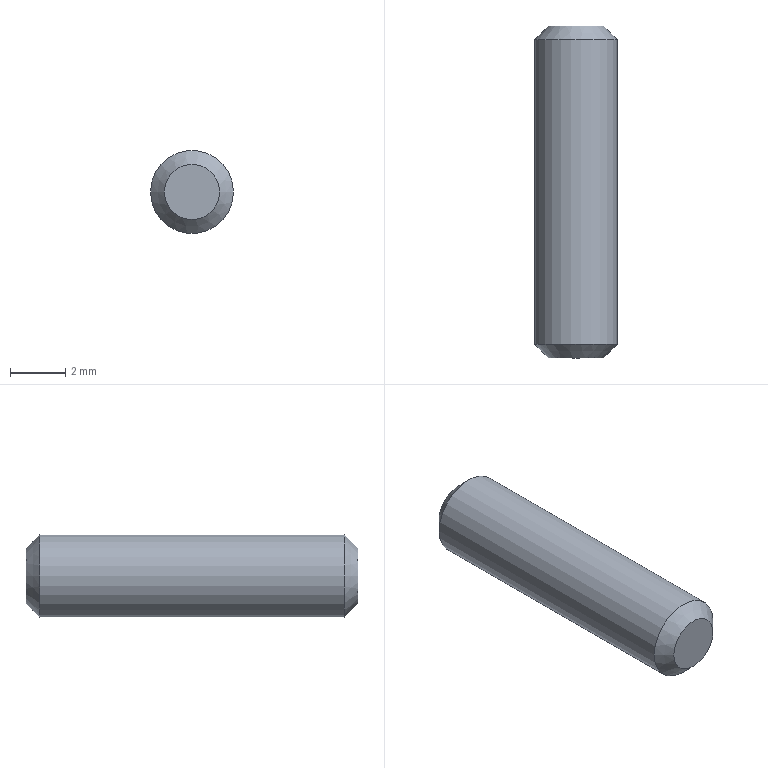Component | NX | PIN_3X12 | 1 solid | 5 faces | box 3 x 12 x 3 mm | volume 83 mm3 | plane 2 | cone 2 | cylinder 1 | commonest cylinder face diameters 3 x1
STEP:
#1=CARTESIAN_POINT('',(0.,0.,0.));
#2=DIRECTION('',(0.,0.,1.));
#3=DIRECTION('',(1.,0.,0.));
#4=AXIS2_PLACEMENT_3D('',#1,#2,#3);
#5=CARTESIAN_POINT('',(380.303,-166.25,-145.));
#6=VERTEX_POINT('',#5);
#7=CARTESIAN_POINT('',(378.803,-166.25,-145.));
#8=DIRECTION('',(0.,-1.,0.));
#9=DIRECTION('',(1.,0.,0.));
#10=AXIS2_PLACEMENT_3D('',#7,#8,#9);
#11=CIRCLE('',#10,1.5);
#12=CARTESIAN_POINT('',(378.803,-177.75,-145.));
#13=DIRECTION('',(0.,1.,0.));
#14=DIRECTION('',(-1.,0.,0.));
#15=AXIS2_PLACEMENT_3D('',#12,#13,#14);
#16=CYLINDRICAL_SURFACE('',#15,1.5);
#17=CARTESIAN_POINT('',(9.425,11.5));
#18=DIRECTION('',(-1.,0.));
#19=VECTOR('',#18,1.);
#20=LINE('',#17,#19);
#21=(GEOMETRIC_REPRESENTATION_CONTEXT(2)PARAMETRIC_REPRESENTATION_CONTEXT()REPRESENTATION_CONTEXT('',''));
#22=DEFINITIONAL_REPRESENTATION('',(#20),#21);
#23=PCURVE('',#16,#22);
#24=CARTESIAN_POINT('',(378.803,-166.25,-145.));
#25=DIRECTION('',(0.,-1.,0.));
#26=DIRECTION('',(1.,0.,0.));
#27=AXIS2_PLACEMENT_3D('',#24,#25,#26);
#28=CONICAL_SURFACE('',#27,1.5,0.7854);
#29=CARTESIAN_POINT('',(0.,0.));
#30=DIRECTION('',(1.,0.));
#31=VECTOR('',#30,1.);
#32=LINE('',#29,#31);
#33=(GEOMETRIC_REPRESENTATION_CONTEXT(2)PARAMETRIC_REPRESENTATION_CONTEXT()REPRESENTATION_CONTEXT('',''));
#34=DEFINITIONAL_REPRESENTATION('',(#32),#33);
#35=PCURVE('',#28,#34);
#36=SURFACE_CURVE('',#11,(#23,#35),.PCURVE_S1.);
#37=EDGE_CURVE('',#6,#6,#36,.T.);
#38=ORIENTED_EDGE('',*,*,#37,.T.);
#39=CARTESIAN_POINT('',(380.303,-177.25,-145.));
#40=VERTEX_POINT('',#39);
#41=CARTESIAN_POINT('',(380.303,-177.25,-145.));
#42=CARTESIAN_POINT('',(380.303,-166.25,-145.));
#43=B_SPLINE_CURVE_WITH_KNOTS('',1,(#41,#42),.UNSPECIFIED.,.F.,.F.,(2,2),(0.5,11.5),.PIECEWISE_BEZIER_KNOTS.);
#44=CARTESIAN_POINT('',(3.142,0.));
#45=DIRECTION('',(0.,1.));
#46=VECTOR('',#45,1.);
#47=LINE('',#44,#46);
#48=(GEOMETRIC_REPRESENTATION_CONTEXT(2)PARAMETRIC_REPRESENTATION_CONTEXT()REPRESENTATION_CONTEXT('',''));
#49=DEFINITIONAL_REPRESENTATION('',(#47),#48);
#50=PCURVE('',#16,#49);
#51=CARTESIAN_POINT('',(9.425,0.));
#52=DIRECTION('',(0.,1.));
#53=VECTOR('',#52,1.);
#54=LINE('',#51,#53);
#55=(GEOMETRIC_REPRESENTATION_CONTEXT(2)PARAMETRIC_REPRESENTATION_CONTEXT()REPRESENTATION_CONTEXT('',''));
#56=DEFINITIONAL_REPRESENTATION('',(#54),#55);
#57=PCURVE('',#16,#56);
#58=SEAM_CURVE('',#43,(#50,#57),.PCURVE_S1.);
#59=EDGE_CURVE('',#40,#6,#58,.T.);
#60=ORIENTED_EDGE('',*,*,#59,.F.);
#61=CARTESIAN_POINT('',(378.803,-177.25,-145.));
#62=DIRECTION('',(0.,1.,0.));
#63=DIRECTION('',(1.,0.,0.));
#64=AXIS2_PLACEMENT_3D('',#61,#62,#63);
#65=CIRCLE('',#64,1.5);
#66=CARTESIAN_POINT('',(3.142,0.5));
#67=DIRECTION('',(1.,0.));
#68=VECTOR('',#67,1.);
#69=LINE('',#66,#68);
#70=(GEOMETRIC_REPRESENTATION_CONTEXT(2)PARAMETRIC_REPRESENTATION_CONTEXT()REPRESENTATION_CONTEXT('',''));
#71=DEFINITIONAL_REPRESENTATION('',(#69),#70);
#72=PCURVE('',#16,#71);
#73=CARTESIAN_POINT('',(378.803,-177.75,-145.));
#74=DIRECTION('',(0.,1.,0.));
#75=DIRECTION('',(-1.,0.,0.));
#76=AXIS2_PLACEMENT_3D('',#73,#74,#75);
#77=CONICAL_SURFACE('',#76,1.,0.7854);
#78=CARTESIAN_POINT('',(3.142,0.5));
#79=DIRECTION('',(1.,0.));
#80=VECTOR('',#79,1.);
#81=LINE('',#78,#80);
#82=(GEOMETRIC_REPRESENTATION_CONTEXT(2)PARAMETRIC_REPRESENTATION_CONTEXT()REPRESENTATION_CONTEXT('',''));
#83=DEFINITIONAL_REPRESENTATION('',(#81),#82);
#84=PCURVE('',#77,#83);
#85=SURFACE_CURVE('',#65,(#72,#84),.PCURVE_S1.);
#86=EDGE_CURVE('',#40,#40,#85,.T.);
#87=ORIENTED_EDGE('',*,*,#86,.T.);
#88=ORIENTED_EDGE('',*,*,#59,.T.);
#89=EDGE_LOOP('',(#38,#60,#87,#88));
#90=FACE_BOUND('',#89,.T.);
#91=ADVANCED_FACE('',(#90),#16,.T.);
#92=CARTESIAN_POINT('',(379.803,-177.75,-145.));
#93=VERTEX_POINT('',#92);
#94=CARTESIAN_POINT('',(378.803,-177.75,-145.));
#95=DIRECTION('',(0.,-1.,0.));
#96=DIRECTION('',(1.,0.,0.));
#97=AXIS2_PLACEMENT_3D('',#94,#95,#96);
#98=CIRCLE('',#97,1.);
#99=CARTESIAN_POINT('',(378.803,-177.75,-145.));
#100=DIRECTION('',(0.,-1.,0.));
#101=DIRECTION('',(1.,0.,0.));
#102=AXIS2_PLACEMENT_3D('',#99,#100,#101);
#103=PLANE('',#102);
#104=CARTESIAN_POINT('',(0.,0.));
#105=DIRECTION('',(1.,0.));
#106=AXIS2_PLACEMENT_2D('',#104,#105);
#107=CIRCLE('',#106,1.);
#108=(GEOMETRIC_REPRESENTATION_CONTEXT(2)PARAMETRIC_REPRESENTATION_CONTEXT()REPRESENTATION_CONTEXT('',''));
#109=DEFINITIONAL_REPRESENTATION('',(#107),#108);
#110=PCURVE('',#103,#109);
#111=CARTESIAN_POINT('',(9.425,0.));
#112=DIRECTION('',(-1.,0.));
#113=VECTOR('',#112,1.);
#114=LINE('',#111,#113);
#115=(GEOMETRIC_REPRESENTATION_CONTEXT(2)PARAMETRIC_REPRESENTATION_CONTEXT()REPRESENTATION_CONTEXT('',''));
#116=DEFINITIONAL_REPRESENTATION('',(#114),#115);
#117=PCURVE('',#77,#116);
#118=SURFACE_CURVE('',#98,(#110,#117),.PCURVE_S1.);
#119=EDGE_CURVE('',#93,#93,#118,.T.);
#120=ORIENTED_EDGE('',*,*,#119,.T.);
#121=EDGE_LOOP('',(#120));
#122=FACE_BOUND('',#121,.T.);
#123=ADVANCED_FACE('',(#122),#103,.T.);
#124=CARTESIAN_POINT('',(379.803,-165.75,-145.));
#125=VERTEX_POINT('',#124);
#126=CARTESIAN_POINT('',(378.803,-165.75,-145.));
#127=DIRECTION('',(0.,1.,0.));
#128=DIRECTION('',(1.,0.,0.));
#129=AXIS2_PLACEMENT_3D('',#126,#127,#128);
#130=CIRCLE('',#129,1.);
#131=CARTESIAN_POINT('',(378.803,-165.75,-145.));
#132=DIRECTION('',(0.,-1.,0.));
#133=DIRECTION('',(1.,0.,0.));
#134=AXIS2_PLACEMENT_3D('',#131,#132,#133);
#135=PLANE('',#134);
#136=CARTESIAN_POINT('',(1.,0.));
#137=CARTESIAN_POINT('',(1.,-1.732));
#138=CARTESIAN_POINT('',(-0.5,-0.866));
#139=CARTESIAN_POINT('',(-2.,-0.));
#140=CARTESIAN_POINT('',(-0.5,0.866));
#141=CARTESIAN_POINT('',(1.,1.732));
#142=CARTESIAN_POINT('',(1.,0.));
#143=(BOUNDED_CURVE()B_SPLINE_CURVE(2,(#136,#137,#138,#139,#140,#141,#142),.UNSPECIFIED.,.T.,.F.)B_SPLINE_CURVE_WITH_KNOTS((1,2,2,2,2,1),(-2.094,0.,2.094,4.189,6.283,8.378),.UNSPECIFIED.)CURVE()GEOMETRIC_REPRESENTATION_ITEM()RATIONAL_B_SPLINE_CURVE((1.,0.5,1.,0.5,1.,0.5,1.))REPRESENTATION_ITEM(''));
#144=(GEOMETRIC_REPRESENTATION_CONTEXT(2)PARAMETRIC_REPRESENTATION_CONTEXT()REPRESENTATION_CONTEXT('',''));
#145=DEFINITIONAL_REPRESENTATION('',(#143),#144);
#146=PCURVE('',#135,#145);
#147=CARTESIAN_POINT('',(6.283,-0.5));
#148=DIRECTION('',(-1.,0.));
#149=VECTOR('',#148,1.);
#150=LINE('',#147,#149);
#151=(GEOMETRIC_REPRESENTATION_CONTEXT(2)PARAMETRIC_REPRESENTATION_CONTEXT()REPRESENTATION_CONTEXT('',''));
#152=DEFINITIONAL_REPRESENTATION('',(#150),#151);
#153=PCURVE('',#28,#152);
#154=SURFACE_CURVE('',#130,(#146,#153),.PCURVE_S1.);
#155=EDGE_CURVE('',#125,#125,#154,.T.);
#156=ORIENTED_EDGE('',*,*,#155,.T.);
#157=EDGE_LOOP('',(#156));
#158=FACE_BOUND('',#157,.T.);
#159=ADVANCED_FACE('',(#158),#135,.F.);
#160=ORIENTED_EDGE('',*,*,#155,.F.);
#161=CARTESIAN_POINT('',(379.803,-165.75,-145.));
#162=CARTESIAN_POINT('',(380.303,-166.25,-145.));
#163=B_SPLINE_CURVE_WITH_KNOTS('',1,(#161,#162),.UNSPECIFIED.,.F.,.F.,(2,2),(-0.7071,0.),.PIECEWISE_BEZIER_KNOTS.);
#164=CARTESIAN_POINT('',(6.283,0.));
#165=DIRECTION('',(0.,1.));
#166=VECTOR('',#165,1.);
#167=LINE('',#164,#166);
#168=(GEOMETRIC_REPRESENTATION_CONTEXT(2)PARAMETRIC_REPRESENTATION_CONTEXT()REPRESENTATION_CONTEXT('',''));
#169=DEFINITIONAL_REPRESENTATION('',(#167),#168);
#170=PCURVE('',#28,#169);
#171=CARTESIAN_POINT('',(0.,0.));
#172=DIRECTION('',(0.,1.));
#173=VECTOR('',#172,1.);
#174=LINE('',#171,#173);
#175=(GEOMETRIC_REPRESENTATION_CONTEXT(2)PARAMETRIC_REPRESENTATION_CONTEXT()REPRESENTATION_CONTEXT('',''));
#176=DEFINITIONAL_REPRESENTATION('',(#174),#175);
#177=PCURVE('',#28,#176);
#178=SEAM_CURVE('',#163,(#170,#177),.PCURVE_S1.);
#179=EDGE_CURVE('',#125,#6,#178,.T.);
#180=ORIENTED_EDGE('',*,*,#179,.T.);
#181=ORIENTED_EDGE('',*,*,#37,.F.);
#182=ORIENTED_EDGE('',*,*,#179,.F.);
#183=EDGE_LOOP('',(#160,#180,#181,#182));
#184=FACE_BOUND('',#183,.T.);
#185=ADVANCED_FACE('',(#184),#28,.T.);
#186=ORIENTED_EDGE('',*,*,#86,.F.);
#187=CARTESIAN_POINT('',(379.803,-177.75,-145.));
#188=CARTESIAN_POINT('',(380.303,-177.25,-145.));
#189=B_SPLINE_CURVE_WITH_KNOTS('',1,(#187,#188),.UNSPECIFIED.,.F.,.F.,(2,2),(0.,0.7071),.PIECEWISE_BEZIER_KNOTS.);
#190=CARTESIAN_POINT('',(3.142,0.));
#191=DIRECTION('',(0.,1.));
#192=VECTOR('',#191,1.);
#193=LINE('',#190,#192);
#194=(GEOMETRIC_REPRESENTATION_CONTEXT(2)PARAMETRIC_REPRESENTATION_CONTEXT()REPRESENTATION_CONTEXT('',''));
#195=DEFINITIONAL_REPRESENTATION('',(#193),#194);
#196=PCURVE('',#77,#195);
#197=CARTESIAN_POINT('',(9.425,0.));
#198=DIRECTION('',(0.,1.));
#199=VECTOR('',#198,1.);
#200=LINE('',#197,#199);
#201=(GEOMETRIC_REPRESENTATION_CONTEXT(2)PARAMETRIC_REPRESENTATION_CONTEXT()REPRESENTATION_CONTEXT('',''));
#202=DEFINITIONAL_REPRESENTATION('',(#200),#201);
#203=PCURVE('',#77,#202);
#204=SEAM_CURVE('',#189,(#196,#203),.PCURVE_S1.);
#205=EDGE_CURVE('',#93,#40,#204,.T.);
#206=ORIENTED_EDGE('',*,*,#205,.F.);
#207=ORIENTED_EDGE('',*,*,#119,.F.);
#208=ORIENTED_EDGE('',*,*,#205,.T.);
#209=EDGE_LOOP('',(#186,#206,#207,#208));
#210=FACE_BOUND('',#209,.T.);
#211=ADVANCED_FACE('',(#210),#77,.T.);
#212=CLOSED_SHELL('',(#91,#123,#159,#185,#211));
#213=MANIFOLD_SOLID_BREP('',#212);
#214=(LENGTH_UNIT()NAMED_UNIT(*)SI_UNIT(.MILLI.,.METRE.));
#215=UNCERTAINTY_MEASURE_WITH_UNIT(LENGTH_MEASURE(0.00001),#214,'','');
#216=(NAMED_UNIT(*)PLANE_ANGLE_UNIT()SI_UNIT($,.RADIAN.));
#217=(NAMED_UNIT(*)SI_UNIT($,.STERADIAN.)SOLID_ANGLE_UNIT());
#218=(GEOMETRIC_REPRESENTATION_CONTEXT(3)GLOBAL_UNCERTAINTY_ASSIGNED_CONTEXT((#215))GLOBAL_UNIT_ASSIGNED_CONTEXT((#214,#216,#217))REPRESENTATION_CONTEXT('',''));
#219=ADVANCED_BREP_SHAPE_REPRESENTATION('',(#4,#213),#218);